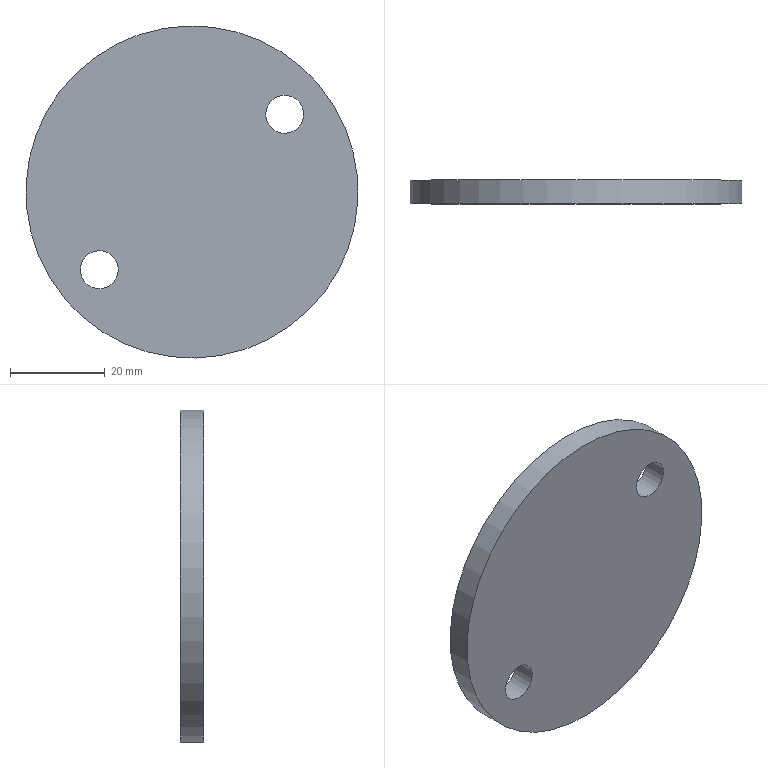Component | NX | MODEL8 | 1 solid | 5 faces | box 70 x 5 x 70 mm | volume 18740 mm3 | cylinder 3 | plane 2 | commonest cylinder face diameters 8 x2 70 x1
STEP:
#1=CARTESIAN_POINT('',(0.,0.,0.));
#2=DIRECTION('',(0.,0.,1.));
#3=DIRECTION('',(1.,0.,0.));
#4=AXIS2_PLACEMENT_3D('',#1,#2,#3);
#5=CARTESIAN_POINT('',(843.53,15.431,-116.584));
#6=VERTEX_POINT('',#5);
#7=CARTESIAN_POINT('',(840.466,15.431,-119.155));
#8=DIRECTION('',(0.,-1.,0.));
#9=DIRECTION('',(0.766,0.,0.6428));
#10=AXIS2_PLACEMENT_3D('',#7,#8,#9);
#11=CIRCLE('',#10,4.);
#12=CARTESIAN_POINT('',(840.466,15.431,-119.155));
#13=DIRECTION('',(0.,1.,0.));
#14=DIRECTION('',(-0.766,0.,-0.6428));
#15=AXIS2_PLACEMENT_3D('',#12,#13,#14);
#16=CYLINDRICAL_SURFACE('',#15,4.);
#17=CARTESIAN_POINT('',(9.425,0.));
#18=DIRECTION('',(-1.,0.));
#19=VECTOR('',#18,1.);
#20=LINE('',#17,#19);
#21=(GEOMETRIC_REPRESENTATION_CONTEXT(2)PARAMETRIC_REPRESENTATION_CONTEXT()REPRESENTATION_CONTEXT('',''));
#22=DEFINITIONAL_REPRESENTATION('',(#20),#21);
#23=PCURVE('',#16,#22);
#24=CARTESIAN_POINT('',(850.233,15.431,-110.96));
#25=DIRECTION('',(0.,-1.,0.));
#26=DIRECTION('',(0.766,0.,0.6428));
#27=AXIS2_PLACEMENT_3D('',#24,#25,#26);
#28=PLANE('',#27);
#29=CARTESIAN_POINT('',(-12.75,-0.));
#30=DIRECTION('',(1.,-0.));
#31=AXIS2_PLACEMENT_2D('',#29,#30);
#32=CIRCLE('',#31,4.);
#33=(GEOMETRIC_REPRESENTATION_CONTEXT(2)PARAMETRIC_REPRESENTATION_CONTEXT()REPRESENTATION_CONTEXT('',''));
#34=DEFINITIONAL_REPRESENTATION('',(#32),#33);
#35=PCURVE('',#28,#34);
#36=SURFACE_CURVE('',#11,(#23,#35),.PCURVE_S1.);
#37=EDGE_CURVE('',#6,#6,#36,.T.);
#38=ORIENTED_EDGE('',*,*,#37,.F.);
#39=CARTESIAN_POINT('',(843.53,20.431,-116.584));
#40=VERTEX_POINT('',#39);
#41=CARTESIAN_POINT('',(843.53,15.431,-116.584));
#42=CARTESIAN_POINT('',(843.53,20.431,-116.584));
#43=B_SPLINE_CURVE_WITH_KNOTS('',1,(#41,#42),.UNSPECIFIED.,.F.,.F.,(2,2),(0.,5.),.PIECEWISE_BEZIER_KNOTS.);
#44=CARTESIAN_POINT('',(9.425,0.));
#45=DIRECTION('',(0.,1.));
#46=VECTOR('',#45,1.);
#47=LINE('',#44,#46);
#48=(GEOMETRIC_REPRESENTATION_CONTEXT(2)PARAMETRIC_REPRESENTATION_CONTEXT()REPRESENTATION_CONTEXT('',''));
#49=DEFINITIONAL_REPRESENTATION('',(#47),#48);
#50=PCURVE('',#16,#49);
#51=CARTESIAN_POINT('',(3.142,0.));
#52=DIRECTION('',(0.,1.));
#53=VECTOR('',#52,1.);
#54=LINE('',#51,#53);
#55=(GEOMETRIC_REPRESENTATION_CONTEXT(2)PARAMETRIC_REPRESENTATION_CONTEXT()REPRESENTATION_CONTEXT('',''));
#56=DEFINITIONAL_REPRESENTATION('',(#54),#55);
#57=PCURVE('',#16,#56);
#58=SEAM_CURVE('',#43,(#50,#57),.PCURVE_S1.);
#59=EDGE_CURVE('',#6,#40,#58,.T.);
#60=ORIENTED_EDGE('',*,*,#59,.T.);
#61=CARTESIAN_POINT('',(840.466,20.431,-119.155));
#62=DIRECTION('',(0.,-1.,0.));
#63=DIRECTION('',(0.766,0.,0.6428));
#64=AXIS2_PLACEMENT_3D('',#61,#62,#63);
#65=CIRCLE('',#64,4.);
#66=CARTESIAN_POINT('',(9.425,5.));
#67=DIRECTION('',(-1.,0.));
#68=VECTOR('',#67,1.);
#69=LINE('',#66,#68);
#70=(GEOMETRIC_REPRESENTATION_CONTEXT(2)PARAMETRIC_REPRESENTATION_CONTEXT()REPRESENTATION_CONTEXT('',''));
#71=DEFINITIONAL_REPRESENTATION('',(#69),#70);
#72=PCURVE('',#16,#71);
#73=CARTESIAN_POINT('',(850.233,20.431,-110.96));
#74=DIRECTION('',(0.,-1.,0.));
#75=DIRECTION('',(0.766,0.,0.6428));
#76=AXIS2_PLACEMENT_3D('',#73,#74,#75);
#77=PLANE('',#76);
#78=CARTESIAN_POINT('',(-12.75,-0.));
#79=DIRECTION('',(1.,-0.));
#80=AXIS2_PLACEMENT_2D('',#78,#79);
#81=CIRCLE('',#80,4.);
#82=(GEOMETRIC_REPRESENTATION_CONTEXT(2)PARAMETRIC_REPRESENTATION_CONTEXT()REPRESENTATION_CONTEXT('',''));
#83=DEFINITIONAL_REPRESENTATION('',(#81),#82);
#84=PCURVE('',#77,#83);
#85=SURFACE_CURVE('',#65,(#72,#84),.PCURVE_S1.);
#86=EDGE_CURVE('',#40,#40,#85,.T.);
#87=ORIENTED_EDGE('',*,*,#86,.T.);
#88=ORIENTED_EDGE('',*,*,#59,.F.);
#89=EDGE_LOOP('',(#38,#60,#87,#88));
#90=FACE_BOUND('',#89,.F.);
#91=ADVANCED_FACE('',(#90),#16,.F.);
#92=CARTESIAN_POINT('',(886.812,15.431,-80.267));
#93=VERTEX_POINT('',#92);
#94=CARTESIAN_POINT('',(860.,15.431,-102.764));
#95=DIRECTION('',(0.,-1.,0.));
#96=DIRECTION('',(0.766,0.,0.6428));
#97=AXIS2_PLACEMENT_3D('',#94,#95,#96);
#98=CIRCLE('',#97,35.);
#99=CARTESIAN_POINT('',(860.,15.431,-102.764));
#100=DIRECTION('',(0.,1.,0.));
#101=DIRECTION('',(-0.766,0.,-0.6428));
#102=AXIS2_PLACEMENT_3D('',#99,#100,#101);
#103=CYLINDRICAL_SURFACE('',#102,35.);
#104=CARTESIAN_POINT('',(9.425,0.));
#105=DIRECTION('',(-1.,0.));
#106=VECTOR('',#105,1.);
#107=LINE('',#104,#106);
#108=(GEOMETRIC_REPRESENTATION_CONTEXT(2)PARAMETRIC_REPRESENTATION_CONTEXT()REPRESENTATION_CONTEXT('',''));
#109=DEFINITIONAL_REPRESENTATION('',(#107),#108);
#110=PCURVE('',#103,#109);
#111=CARTESIAN_POINT('',(12.75,0.));
#112=DIRECTION('',(1.,-0.));
#113=AXIS2_PLACEMENT_2D('',#111,#112);
#114=CIRCLE('',#113,35.);
#115=(GEOMETRIC_REPRESENTATION_CONTEXT(2)PARAMETRIC_REPRESENTATION_CONTEXT()REPRESENTATION_CONTEXT('',''));
#116=DEFINITIONAL_REPRESENTATION('',(#114),#115);
#117=PCURVE('',#28,#116);
#118=SURFACE_CURVE('',#98,(#110,#117),.PCURVE_S1.);
#119=EDGE_CURVE('',#93,#93,#118,.T.);
#120=ORIENTED_EDGE('',*,*,#119,.F.);
#121=CARTESIAN_POINT('',(886.812,20.431,-80.267));
#122=VERTEX_POINT('',#121);
#123=CARTESIAN_POINT('',(886.812,15.431,-80.267));
#124=CARTESIAN_POINT('',(886.812,20.431,-80.267));
#125=B_SPLINE_CURVE_WITH_KNOTS('',1,(#123,#124),.UNSPECIFIED.,.F.,.F.,(2,2),(0.,5.),.PIECEWISE_BEZIER_KNOTS.);
#126=CARTESIAN_POINT('',(9.425,0.));
#127=DIRECTION('',(0.,1.));
#128=VECTOR('',#127,1.);
#129=LINE('',#126,#128);
#130=(GEOMETRIC_REPRESENTATION_CONTEXT(2)PARAMETRIC_REPRESENTATION_CONTEXT()REPRESENTATION_CONTEXT('',''));
#131=DEFINITIONAL_REPRESENTATION('',(#129),#130);
#132=PCURVE('',#103,#131);
#133=CARTESIAN_POINT('',(3.142,0.));
#134=DIRECTION('',(0.,1.));
#135=VECTOR('',#134,1.);
#136=LINE('',#133,#135);
#137=(GEOMETRIC_REPRESENTATION_CONTEXT(2)PARAMETRIC_REPRESENTATION_CONTEXT()REPRESENTATION_CONTEXT('',''));
#138=DEFINITIONAL_REPRESENTATION('',(#136),#137);
#139=PCURVE('',#103,#138);
#140=SEAM_CURVE('',#125,(#132,#139),.PCURVE_S1.);
#141=EDGE_CURVE('',#93,#122,#140,.T.);
#142=ORIENTED_EDGE('',*,*,#141,.T.);
#143=CARTESIAN_POINT('',(860.,20.431,-102.764));
#144=DIRECTION('',(0.,-1.,0.));
#145=DIRECTION('',(0.766,0.,0.6428));
#146=AXIS2_PLACEMENT_3D('',#143,#144,#145);
#147=CIRCLE('',#146,35.);
#148=CARTESIAN_POINT('',(9.425,5.));
#149=DIRECTION('',(-1.,0.));
#150=VECTOR('',#149,1.);
#151=LINE('',#148,#150);
#152=(GEOMETRIC_REPRESENTATION_CONTEXT(2)PARAMETRIC_REPRESENTATION_CONTEXT()REPRESENTATION_CONTEXT('',''));
#153=DEFINITIONAL_REPRESENTATION('',(#151),#152);
#154=PCURVE('',#103,#153);
#155=CARTESIAN_POINT('',(12.75,0.));
#156=DIRECTION('',(1.,-0.));
#157=AXIS2_PLACEMENT_2D('',#155,#156);
#158=CIRCLE('',#157,35.);
#159=(GEOMETRIC_REPRESENTATION_CONTEXT(2)PARAMETRIC_REPRESENTATION_CONTEXT()REPRESENTATION_CONTEXT('',''));
#160=DEFINITIONAL_REPRESENTATION('',(#158),#159);
#161=PCURVE('',#77,#160);
#162=SURFACE_CURVE('',#147,(#154,#161),.PCURVE_S1.);
#163=EDGE_CURVE('',#122,#122,#162,.T.);
#164=ORIENTED_EDGE('',*,*,#163,.T.);
#165=ORIENTED_EDGE('',*,*,#141,.F.);
#166=EDGE_LOOP('',(#120,#142,#164,#165));
#167=FACE_BOUND('',#166,.T.);
#168=ADVANCED_FACE('',(#167),#103,.T.);
#169=CARTESIAN_POINT('',(876.47,15.431,-88.944));
#170=VERTEX_POINT('',#169);
#171=CARTESIAN_POINT('',(879.534,15.431,-86.373));
#172=DIRECTION('',(0.,1.,0.));
#173=DIRECTION('',(-0.766,0.,-0.6428));
#174=AXIS2_PLACEMENT_3D('',#171,#172,#173);
#175=CIRCLE('',#174,4.);
#176=CARTESIAN_POINT('',(879.534,15.431,-86.373));
#177=DIRECTION('',(0.,1.,0.));
#178=DIRECTION('',(-0.766,0.,-0.6428));
#179=AXIS2_PLACEMENT_3D('',#176,#177,#178);
#180=CYLINDRICAL_SURFACE('',#179,4.);
#181=CARTESIAN_POINT('',(0.,0.));
#182=DIRECTION('',(1.,0.));
#183=VECTOR('',#182,1.);
#184=LINE('',#181,#183);
#185=(GEOMETRIC_REPRESENTATION_CONTEXT(2)PARAMETRIC_REPRESENTATION_CONTEXT()REPRESENTATION_CONTEXT('',''));
#186=DEFINITIONAL_REPRESENTATION('',(#184),#185);
#187=PCURVE('',#180,#186);
#188=CARTESIAN_POINT('',(34.25,0.));
#189=CARTESIAN_POINT('',(34.25,6.928));
#190=CARTESIAN_POINT('',(40.25,3.464));
#191=CARTESIAN_POINT('',(46.25,0.));
#192=CARTESIAN_POINT('',(40.25,-3.464));
#193=CARTESIAN_POINT('',(34.25,-6.928));
#194=CARTESIAN_POINT('',(34.25,0.));
#195=(BOUNDED_CURVE()B_SPLINE_CURVE(2,(#188,#189,#190,#191,#192,#193,#194),.UNSPECIFIED.,.T.,.F.)B_SPLINE_CURVE_WITH_KNOTS((1,2,2,2,2,1),(-2.094,0.,2.094,4.189,6.283,8.378),.UNSPECIFIED.)CURVE()GEOMETRIC_REPRESENTATION_ITEM()RATIONAL_B_SPLINE_CURVE((1.,0.5,1.,0.5,1.,0.5,1.))REPRESENTATION_ITEM(''));
#196=(GEOMETRIC_REPRESENTATION_CONTEXT(2)PARAMETRIC_REPRESENTATION_CONTEXT()REPRESENTATION_CONTEXT('',''));
#197=DEFINITIONAL_REPRESENTATION('',(#195),#196);
#198=PCURVE('',#28,#197);
#199=SURFACE_CURVE('',#175,(#187,#198),.PCURVE_S1.);
#200=EDGE_CURVE('',#170,#170,#199,.T.);
#201=ORIENTED_EDGE('',*,*,#200,.T.);
#202=CARTESIAN_POINT('',(876.47,20.431,-88.944));
#203=VERTEX_POINT('',#202);
#204=CARTESIAN_POINT('',(876.47,15.431,-88.944));
#205=CARTESIAN_POINT('',(876.47,20.431,-88.944));
#206=B_SPLINE_CURVE_WITH_KNOTS('',1,(#204,#205),.UNSPECIFIED.,.F.,.F.,(2,2),(0.,5.),.PIECEWISE_BEZIER_KNOTS.);
#207=CARTESIAN_POINT('',(6.283,0.));
#208=DIRECTION('',(0.,1.));
#209=VECTOR('',#208,1.);
#210=LINE('',#207,#209);
#211=(GEOMETRIC_REPRESENTATION_CONTEXT(2)PARAMETRIC_REPRESENTATION_CONTEXT()REPRESENTATION_CONTEXT('',''));
#212=DEFINITIONAL_REPRESENTATION('',(#210),#211);
#213=PCURVE('',#180,#212);
#214=CARTESIAN_POINT('',(0.,0.));
#215=DIRECTION('',(0.,1.));
#216=VECTOR('',#215,1.);
#217=LINE('',#214,#216);
#218=(GEOMETRIC_REPRESENTATION_CONTEXT(2)PARAMETRIC_REPRESENTATION_CONTEXT()REPRESENTATION_CONTEXT('',''));
#219=DEFINITIONAL_REPRESENTATION('',(#217),#218);
#220=PCURVE('',#180,#219);
#221=SEAM_CURVE('',#206,(#213,#220),.PCURVE_S1.);
#222=EDGE_CURVE('',#170,#203,#221,.T.);
#223=ORIENTED_EDGE('',*,*,#222,.T.);
#224=CARTESIAN_POINT('',(879.534,20.431,-86.373));
#225=DIRECTION('',(0.,1.,0.));
#226=DIRECTION('',(-0.766,0.,-0.6428));
#227=AXIS2_PLACEMENT_3D('',#224,#225,#226);
#228=CIRCLE('',#227,4.);
#229=CARTESIAN_POINT('',(0.,5.));
#230=DIRECTION('',(1.,0.));
#231=VECTOR('',#230,1.);
#232=LINE('',#229,#231);
#233=(GEOMETRIC_REPRESENTATION_CONTEXT(2)PARAMETRIC_REPRESENTATION_CONTEXT()REPRESENTATION_CONTEXT('',''));
#234=DEFINITIONAL_REPRESENTATION('',(#232),#233);
#235=PCURVE('',#180,#234);
#236=CARTESIAN_POINT('',(34.25,0.));
#237=CARTESIAN_POINT('',(34.25,6.928));
#238=CARTESIAN_POINT('',(40.25,3.464));
#239=CARTESIAN_POINT('',(46.25,0.));
#240=CARTESIAN_POINT('',(40.25,-3.464));
#241=CARTESIAN_POINT('',(34.25,-6.928));
#242=CARTESIAN_POINT('',(34.25,0.));
#243=(BOUNDED_CURVE()B_SPLINE_CURVE(2,(#236,#237,#238,#239,#240,#241,#242),.UNSPECIFIED.,.T.,.F.)B_SPLINE_CURVE_WITH_KNOTS((1,2,2,2,2,1),(-2.094,0.,2.094,4.189,6.283,8.378),.UNSPECIFIED.)CURVE()GEOMETRIC_REPRESENTATION_ITEM()RATIONAL_B_SPLINE_CURVE((1.,0.5,1.,0.5,1.,0.5,1.))REPRESENTATION_ITEM(''));
#244=(GEOMETRIC_REPRESENTATION_CONTEXT(2)PARAMETRIC_REPRESENTATION_CONTEXT()REPRESENTATION_CONTEXT('',''));
#245=DEFINITIONAL_REPRESENTATION('',(#243),#244);
#246=PCURVE('',#77,#245);
#247=SURFACE_CURVE('',#228,(#235,#246),.PCURVE_S1.);
#248=EDGE_CURVE('',#203,#203,#247,.T.);
#249=ORIENTED_EDGE('',*,*,#248,.F.);
#250=ORIENTED_EDGE('',*,*,#222,.F.);
#251=EDGE_LOOP('',(#201,#223,#249,#250));
#252=FACE_BOUND('',#251,.F.);
#253=ADVANCED_FACE('',(#252),#180,.F.);
#254=ORIENTED_EDGE('',*,*,#119,.T.);
#255=EDGE_LOOP('',(#254));
#256=FACE_BOUND('',#255,.T.);
#257=ORIENTED_EDGE('',*,*,#37,.F.);
#258=EDGE_LOOP('',(#257));
#259=FACE_BOUND('',#258,.T.);
#260=ORIENTED_EDGE('',*,*,#200,.T.);
#261=EDGE_LOOP('',(#260));
#262=FACE_BOUND('',#261,.T.);
#263=ADVANCED_FACE('',(#256,#259,#262),#28,.T.);
#264=ORIENTED_EDGE('',*,*,#163,.F.);
#265=EDGE_LOOP('',(#264));
#266=FACE_BOUND('',#265,.T.);
#267=ORIENTED_EDGE('',*,*,#86,.T.);
#268=EDGE_LOOP('',(#267));
#269=FACE_BOUND('',#268,.T.);
#270=ORIENTED_EDGE('',*,*,#248,.F.);
#271=EDGE_LOOP('',(#270));
#272=FACE_BOUND('',#271,.T.);
#273=ADVANCED_FACE('',(#266,#269,#272),#77,.F.);
#274=CLOSED_SHELL('',(#91,#168,#253,#263,#273));
#275=MANIFOLD_SOLID_BREP('',#274);
#276=(LENGTH_UNIT()NAMED_UNIT(*)SI_UNIT(.MILLI.,.METRE.));
#277=UNCERTAINTY_MEASURE_WITH_UNIT(LENGTH_MEASURE(0.00001),#276,'','');
#278=(NAMED_UNIT(*)PLANE_ANGLE_UNIT()SI_UNIT($,.RADIAN.));
#279=(NAMED_UNIT(*)SI_UNIT($,.STERADIAN.)SOLID_ANGLE_UNIT());
#280=(GEOMETRIC_REPRESENTATION_CONTEXT(3)GLOBAL_UNCERTAINTY_ASSIGNED_CONTEXT((#277))GLOBAL_UNIT_ASSIGNED_CONTEXT((#276,#278,#279))REPRESENTATION_CONTEXT('',''));
#281=ADVANCED_BREP_SHAPE_REPRESENTATION('',(#4,#275),#280);